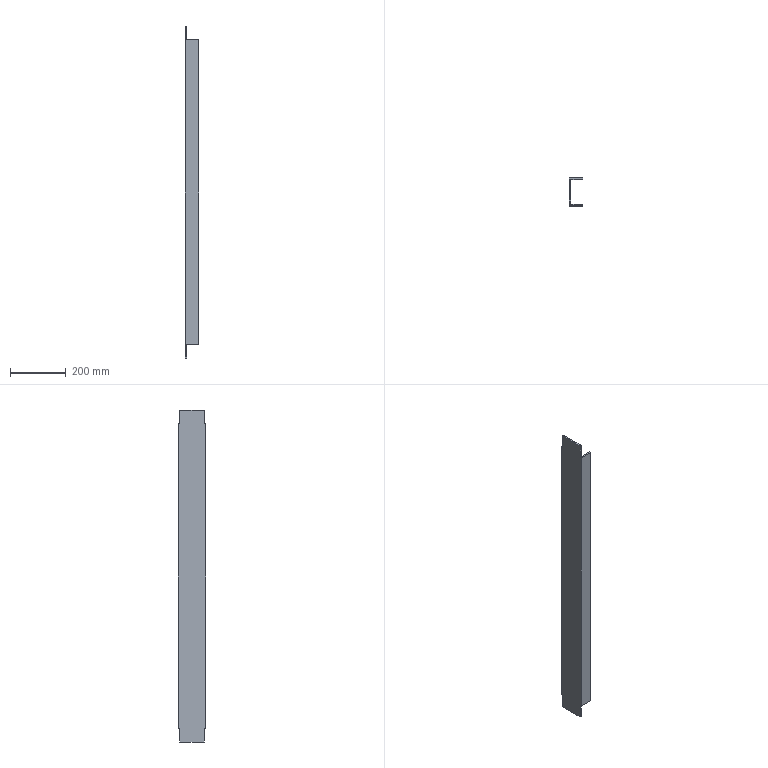Component | SolidWorks | 07ResistorBaseI-1 | 1 solid | 26 faces | box 48 x 100 x 1189 mm | volume 1154519 mm3 | plane 18 | cylinder 8 | commonest cylinder face diameters 12 x8
build123d program:
from build123d import *

# Parameters (mm, degrees)
EXTRUDE_THIN1_DEPTH            = 1189
SKETCH2_W                      = 48
SKETCH2_H                      = 50
CUT_EXTRUDE1_DEPTH             = 5.5
SKETCH3_W                      = 48
SKETCH3_H                      = 50
CUT_EXTRUDE2_DEPTH             = 5.5
F_12_0_12_DIAMETER_HOLE1_D     = 12
F_12_0_12_DIAMETER_HOLE1_DEPTH = 5.5


with BuildPart() as part:
    # Sketch1 → Extrude-Thin1 (new body)
    with BuildSketch(Plane.XY):
        Polygon((48, 0), (0, 0), (0, 100), (48, 100), (48, 94.5), (5.5, 94.5), (5.5, 5.5), (48, 5.5), align=None)
    extrude(amount=EXTRUDE_THIN1_DEPTH)

    # Sketch2 → Cut-Extrude1 (cut)
    with BuildSketch(Plane(origin=(0, 100, 0), x_dir=(1, 0, 0), z_dir=(0, 1, 0))):
        with Locations((24, -1164)):
            Rectangle(SKETCH2_W, SKETCH2_H)
        with Locations((24, -25)):
            Rectangle(SKETCH2_W, SKETCH2_H)
    extrude(amount=-CUT_EXTRUDE1_DEPTH, mode=Mode.SUBTRACT)

    # Sketch3 → Cut-Extrude2 (cut)
    with BuildSketch(Plane.XZ):
        with Locations((24, 25)):
            Rectangle(SKETCH3_W, SKETCH3_H)
        with Locations((24, 1164)):
            Rectangle(SKETCH3_W, SKETCH3_H)
    extrude(amount=-CUT_EXTRUDE2_DEPTH, mode=Mode.SUBTRACT)

    # 12.0 _12_ Diameter Hole1
    with Locations(Plane(origin=(0, 100, 0), x_dir=(-1, 0, 0), z_dir=(0, 1, 0))):
        with Locations((-25, 529.5), (-25, 659.5), (-25, 919.5), (-25, 269.5)):
            Hole(F_12_0_12_DIAMETER_HOLE1_D / 2, depth=F_12_0_12_DIAMETER_HOLE1_DEPTH)


solid = part.part

# Placed as in the assembly
solid = solid.moved(Location((2053.973, -139.54, 42.607), (0, 0, 0)))
STEP:
#1=CARTESIAN_POINT('',(81.849,-1.773,22.288));
#2=VERTEX_POINT('',#1);
#3=CARTESIAN_POINT('',(81.849,-1.773,22.76));
#4=VERTEX_POINT('',#3);
#5=CARTESIAN_POINT('',(81.849,-1.773,22.524));
#6=DIRECTION('',(0.,1.,0.));
#7=DIRECTION('',(0.,0.,1.));
#8=AXIS2_PLACEMENT_3D('',#5,#6,#7);
#9=CIRCLE('',#8,0.2362);
#10=EDGE_CURVE('',#2,#4,#9,.T.);
#11=ORIENTED_EDGE('',*,*,#10,.F.);
#12=CARTESIAN_POINT('',(81.849,-1.557,22.288));
#13=VERTEX_POINT('',#12);
#14=CARTESIAN_POINT('',(81.849,-1.557,22.288));
#15=DIRECTION('',(0.,1.,0.));
#16=VECTOR('',#15,39.37);
#17=LINE('',#14,#16);
#18=EDGE_CURVE('',#2,#13,#17,.T.);
#19=ORIENTED_EDGE('',*,*,#18,.T.);
#20=CARTESIAN_POINT('',(81.849,-1.557,22.76));
#21=VERTEX_POINT('',#20);
#22=CARTESIAN_POINT('',(81.849,-1.557,22.524));
#23=DIRECTION('',(0.,1.,0.));
#24=DIRECTION('',(0.,0.,1.));
#25=AXIS2_PLACEMENT_3D('',#22,#23,#24);
#26=CIRCLE('',#25,0.2362);
#27=EDGE_CURVE('',#13,#21,#26,.T.);
#28=ORIENTED_EDGE('',*,*,#27,.T.);
#29=CARTESIAN_POINT('',(81.849,-1.557,22.76));
#30=DIRECTION('',(0.,1.,0.));
#31=VECTOR('',#30,39.37);
#32=LINE('',#29,#31);
#33=EDGE_CURVE('',#4,#21,#32,.T.);
#34=ORIENTED_EDGE('',*,*,#33,.F.);
#35=EDGE_LOOP('',(#11,#19,#28,#34));
#36=FACE_OUTER_BOUND('',#35,.T.);
#37=CARTESIAN_POINT('',(81.849,-1.557,22.524));
#38=DIRECTION('',(0.,1.,0.));
#39=DIRECTION('',(0.,0.,1.));
#40=AXIS2_PLACEMENT_3D('',#37,#38,#39);
#41=CYLINDRICAL_SURFACE('',#40,0.2362);
#42=ADVANCED_FACE('',(#36),#41,.F.);
#43=CARTESIAN_POINT('',(81.849,-1.773,27.406));
#44=VERTEX_POINT('',#43);
#45=CARTESIAN_POINT('',(81.849,-1.773,27.878));
#46=VERTEX_POINT('',#45);
#47=CARTESIAN_POINT('',(81.849,-1.773,27.642));
#48=DIRECTION('',(0.,1.,0.));
#49=DIRECTION('',(0.,0.,1.));
#50=AXIS2_PLACEMENT_3D('',#47,#48,#49);
#51=CIRCLE('',#50,0.2362);
#52=EDGE_CURVE('',#44,#46,#51,.T.);
#53=ORIENTED_EDGE('',*,*,#52,.F.);
#54=CARTESIAN_POINT('',(81.849,-1.557,27.406));
#55=VERTEX_POINT('',#54);
#56=CARTESIAN_POINT('',(81.849,-1.557,27.406));
#57=DIRECTION('',(0.,1.,0.));
#58=VECTOR('',#57,39.37);
#59=LINE('',#56,#58);
#60=EDGE_CURVE('',#44,#55,#59,.T.);
#61=ORIENTED_EDGE('',*,*,#60,.T.);
#62=CARTESIAN_POINT('',(81.849,-1.557,27.878));
#63=VERTEX_POINT('',#62);
#64=CARTESIAN_POINT('',(81.849,-1.557,27.642));
#65=DIRECTION('',(0.,1.,0.));
#66=DIRECTION('',(0.,0.,1.));
#67=AXIS2_PLACEMENT_3D('',#64,#65,#66);
#68=CIRCLE('',#67,0.2362);
#69=EDGE_CURVE('',#55,#63,#68,.T.);
#70=ORIENTED_EDGE('',*,*,#69,.T.);
#71=CARTESIAN_POINT('',(81.849,-1.557,27.878));
#72=DIRECTION('',(0.,1.,0.));
#73=VECTOR('',#72,39.37);
#74=LINE('',#71,#73);
#75=EDGE_CURVE('',#46,#63,#74,.T.);
#76=ORIENTED_EDGE('',*,*,#75,.F.);
#77=EDGE_LOOP('',(#53,#61,#70,#76));
#78=FACE_OUTER_BOUND('',#77,.T.);
#79=CARTESIAN_POINT('',(81.849,-1.557,27.642));
#80=DIRECTION('',(0.,1.,0.));
#81=DIRECTION('',(0.,0.,1.));
#82=AXIS2_PLACEMENT_3D('',#79,#80,#81);
#83=CYLINDRICAL_SURFACE('',#82,0.2362);
#84=ADVANCED_FACE('',(#78),#83,.F.);
#85=CARTESIAN_POINT('',(81.849,-1.773,37.642));
#86=VERTEX_POINT('',#85);
#87=CARTESIAN_POINT('',(81.849,-1.773,38.114));
#88=VERTEX_POINT('',#87);
#89=CARTESIAN_POINT('',(81.849,-1.773,37.878));
#90=DIRECTION('',(0.,1.,0.));
#91=DIRECTION('',(0.,0.,1.));
#92=AXIS2_PLACEMENT_3D('',#89,#90,#91);
#93=CIRCLE('',#92,0.2362);
#94=EDGE_CURVE('',#86,#88,#93,.T.);
#95=ORIENTED_EDGE('',*,*,#94,.F.);
#96=CARTESIAN_POINT('',(81.849,-1.557,37.642));
#97=VERTEX_POINT('',#96);
#98=CARTESIAN_POINT('',(81.849,-1.557,37.642));
#99=DIRECTION('',(0.,1.,0.));
#100=VECTOR('',#99,39.37);
#101=LINE('',#98,#100);
#102=EDGE_CURVE('',#86,#97,#101,.T.);
#103=ORIENTED_EDGE('',*,*,#102,.T.);
#104=CARTESIAN_POINT('',(81.849,-1.557,38.114));
#105=VERTEX_POINT('',#104);
#106=CARTESIAN_POINT('',(81.849,-1.557,37.878));
#107=DIRECTION('',(0.,1.,0.));
#108=DIRECTION('',(0.,0.,1.));
#109=AXIS2_PLACEMENT_3D('',#106,#107,#108);
#110=CIRCLE('',#109,0.2362);
#111=EDGE_CURVE('',#97,#105,#110,.T.);
#112=ORIENTED_EDGE('',*,*,#111,.T.);
#113=CARTESIAN_POINT('',(81.849,-1.557,38.114));
#114=DIRECTION('',(0.,1.,0.));
#115=VECTOR('',#114,39.37);
#116=LINE('',#113,#115);
#117=EDGE_CURVE('',#88,#105,#116,.T.);
#118=ORIENTED_EDGE('',*,*,#117,.F.);
#119=EDGE_LOOP('',(#95,#103,#112,#118));
#120=FACE_OUTER_BOUND('',#119,.T.);
#121=CARTESIAN_POINT('',(81.849,-1.557,37.878));
#122=DIRECTION('',(0.,1.,0.));
#123=DIRECTION('',(0.,0.,1.));
#124=AXIS2_PLACEMENT_3D('',#121,#122,#123);
#125=CYLINDRICAL_SURFACE('',#124,0.2362);
#126=ADVANCED_FACE('',(#120),#125,.F.);
#127=CARTESIAN_POINT('',(81.849,-1.773,12.051));
#128=VERTEX_POINT('',#127);
#129=CARTESIAN_POINT('',(81.849,-1.773,12.524));
#130=VERTEX_POINT('',#129);
#131=CARTESIAN_POINT('',(81.849,-1.773,12.288));
#132=DIRECTION('',(0.,1.,0.));
#133=DIRECTION('',(0.,0.,1.));
#134=AXIS2_PLACEMENT_3D('',#131,#132,#133);
#135=CIRCLE('',#134,0.2362);
#136=EDGE_CURVE('',#128,#130,#135,.T.);
#137=ORIENTED_EDGE('',*,*,#136,.F.);
#138=CARTESIAN_POINT('',(81.849,-1.557,12.051));
#139=VERTEX_POINT('',#138);
#140=CARTESIAN_POINT('',(81.849,-1.557,12.051));
#141=DIRECTION('',(0.,1.,0.));
#142=VECTOR('',#141,39.37);
#143=LINE('',#140,#142);
#144=EDGE_CURVE('',#128,#139,#143,.T.);
#145=ORIENTED_EDGE('',*,*,#144,.T.);
#146=CARTESIAN_POINT('',(81.849,-1.557,12.524));
#147=VERTEX_POINT('',#146);
#148=CARTESIAN_POINT('',(81.849,-1.557,12.288));
#149=DIRECTION('',(0.,1.,0.));
#150=DIRECTION('',(0.,0.,1.));
#151=AXIS2_PLACEMENT_3D('',#148,#149,#150);
#152=CIRCLE('',#151,0.2362);
#153=EDGE_CURVE('',#139,#147,#152,.T.);
#154=ORIENTED_EDGE('',*,*,#153,.T.);
#155=CARTESIAN_POINT('',(81.849,-1.557,12.524));
#156=DIRECTION('',(0.,1.,0.));
#157=VECTOR('',#156,39.37);
#158=LINE('',#155,#157);
#159=EDGE_CURVE('',#130,#147,#158,.T.);
#160=ORIENTED_EDGE('',*,*,#159,.F.);
#161=EDGE_LOOP('',(#137,#145,#154,#160));
#162=FACE_OUTER_BOUND('',#161,.T.);
#163=CARTESIAN_POINT('',(81.849,-1.557,12.288));
#164=DIRECTION('',(0.,1.,0.));
#165=DIRECTION('',(0.,0.,1.));
#166=AXIS2_PLACEMENT_3D('',#163,#164,#165);
#167=CYLINDRICAL_SURFACE('',#166,0.2362);
#168=ADVANCED_FACE('',(#162),#167,.F.);
#169=CARTESIAN_POINT('',(80.865,-5.277,48.488));
#170=VERTEX_POINT('',#169);
#171=CARTESIAN_POINT('',(81.082,-5.277,48.488));
#172=VERTEX_POINT('',#171);
#173=CARTESIAN_POINT('',(82.755,-5.277,48.488));
#174=DIRECTION('',(1.,-0.,0.));
#175=VECTOR('',#174,39.37);
#176=LINE('',#173,#175);
#177=EDGE_CURVE('',#170,#172,#176,.T.);
#178=ORIENTED_EDGE('',*,*,#177,.T.);
#179=CARTESIAN_POINT('',(81.082,-1.773,48.488));
#180=VERTEX_POINT('',#179);
#181=CARTESIAN_POINT('',(81.082,-5.494,48.488));
#182=DIRECTION('',(0.,1.,0.));
#183=VECTOR('',#182,39.37);
#184=LINE('',#181,#183);
#185=EDGE_CURVE('',#172,#180,#184,.T.);
#186=ORIENTED_EDGE('',*,*,#185,.T.);
#187=CARTESIAN_POINT('',(80.865,-1.773,48.488));
#188=VERTEX_POINT('',#187);
#189=CARTESIAN_POINT('',(82.755,-1.773,48.488));
#190=DIRECTION('',(1.,0.,0.));
#191=VECTOR('',#190,39.37);
#192=LINE('',#189,#191);
#193=EDGE_CURVE('',#188,#180,#192,.T.);
#194=ORIENTED_EDGE('',*,*,#193,.F.);
#195=CARTESIAN_POINT('',(80.865,-5.494,48.488));
#196=DIRECTION('',(0.,1.,0.));
#197=VECTOR('',#196,39.37);
#198=LINE('',#195,#197);
#199=EDGE_CURVE('',#170,#188,#198,.T.);
#200=ORIENTED_EDGE('',*,*,#199,.F.);
#201=EDGE_LOOP('',(#178,#186,#194,#200));
#202=FACE_OUTER_BOUND('',#201,.T.);
#203=CARTESIAN_POINT('',(82.755,-1.773,48.488));
#204=DIRECTION('',(0.,0.,-1.));
#205=DIRECTION('',(-1.,0.,0.));
#206=AXIS2_PLACEMENT_3D('',#203,#204,#205);
#207=PLANE('',#206);
#208=ADVANCED_FACE('',(#202),#207,.F.);
#209=CARTESIAN_POINT('',(81.082,-5.277,1.677));
#210=VERTEX_POINT('',#209);
#211=CARTESIAN_POINT('',(81.082,-1.773,1.677));
#212=VERTEX_POINT('',#211);
#213=CARTESIAN_POINT('',(81.082,-5.494,1.677));
#214=DIRECTION('',(0.,1.,0.));
#215=VECTOR('',#214,39.37);
#216=LINE('',#213,#215);
#217=EDGE_CURVE('',#210,#212,#216,.T.);
#218=ORIENTED_EDGE('',*,*,#217,.F.);
#219=CARTESIAN_POINT('',(80.865,-5.277,1.677));
#220=VERTEX_POINT('',#219);
#221=CARTESIAN_POINT('',(82.755,-5.277,1.677));
#222=DIRECTION('',(-1.,0.,0.));
#223=VECTOR('',#222,39.37);
#224=LINE('',#221,#223);
#225=EDGE_CURVE('',#210,#220,#224,.T.);
#226=ORIENTED_EDGE('',*,*,#225,.T.);
#227=CARTESIAN_POINT('',(80.865,-1.773,1.677));
#228=VERTEX_POINT('',#227);
#229=CARTESIAN_POINT('',(80.865,-5.494,1.677));
#230=DIRECTION('',(0.,1.,0.));
#231=VECTOR('',#230,39.37);
#232=LINE('',#229,#231);
#233=EDGE_CURVE('',#220,#228,#232,.T.);
#234=ORIENTED_EDGE('',*,*,#233,.T.);
#235=CARTESIAN_POINT('',(82.755,-1.773,1.677));
#236=DIRECTION('',(1.,0.,0.));
#237=VECTOR('',#236,39.37);
#238=LINE('',#235,#237);
#239=EDGE_CURVE('',#228,#212,#238,.T.);
#240=ORIENTED_EDGE('',*,*,#239,.T.);
#241=EDGE_LOOP('',(#218,#226,#234,#240));
#242=FACE_OUTER_BOUND('',#241,.T.);
#243=CARTESIAN_POINT('',(82.755,-1.773,1.677));
#244=DIRECTION('',(0.,0.,-1.));
#245=DIRECTION('',(-1.,0.,0.));
#246=AXIS2_PLACEMENT_3D('',#243,#244,#245);
#247=PLANE('',#246);
#248=ADVANCED_FACE('',(#242),#247,.T.);
#249=CARTESIAN_POINT('',(81.849,-1.773,22.524));
#250=DIRECTION('',(0.,1.,0.));
#251=DIRECTION('',(0.,0.,1.));
#252=AXIS2_PLACEMENT_3D('',#249,#250,#251);
#253=CIRCLE('',#252,0.2362);
#254=EDGE_CURVE('',#4,#2,#253,.T.);
#255=ORIENTED_EDGE('',*,*,#254,.T.);
#256=ORIENTED_EDGE('',*,*,#10,.T.);
#257=EDGE_LOOP('',(#255,#256));
#258=FACE_BOUND('',#257,.T.);
#259=CARTESIAN_POINT('',(81.849,-1.773,27.642));
#260=DIRECTION('',(0.,1.,0.));
#261=DIRECTION('',(0.,0.,1.));
#262=AXIS2_PLACEMENT_3D('',#259,#260,#261);
#263=CIRCLE('',#262,0.2362);
#264=EDGE_CURVE('',#46,#44,#263,.T.);
#265=ORIENTED_EDGE('',*,*,#264,.T.);
#266=ORIENTED_EDGE('',*,*,#52,.T.);
#267=EDGE_LOOP('',(#265,#266));
#268=FACE_BOUND('',#267,.T.);
#269=CARTESIAN_POINT('',(81.849,-1.773,37.878));
#270=DIRECTION('',(0.,1.,0.));
#271=DIRECTION('',(0.,0.,1.));
#272=AXIS2_PLACEMENT_3D('',#269,#270,#271);
#273=CIRCLE('',#272,0.2362);
#274=EDGE_CURVE('',#88,#86,#273,.T.);
#275=ORIENTED_EDGE('',*,*,#274,.T.);
#276=ORIENTED_EDGE('',*,*,#94,.T.);
#277=EDGE_LOOP('',(#275,#276));
#278=FACE_BOUND('',#277,.T.);
#279=CARTESIAN_POINT('',(81.849,-1.773,12.288));
#280=DIRECTION('',(0.,1.,0.));
#281=DIRECTION('',(0.,0.,1.));
#282=AXIS2_PLACEMENT_3D('',#279,#280,#281);
#283=CIRCLE('',#282,0.2362);
#284=EDGE_CURVE('',#130,#128,#283,.T.);
#285=ORIENTED_EDGE('',*,*,#284,.T.);
#286=ORIENTED_EDGE('',*,*,#136,.T.);
#287=EDGE_LOOP('',(#285,#286));
#288=FACE_BOUND('',#287,.T.);
#289=CARTESIAN_POINT('',(81.082,-1.773,46.52));
#290=VERTEX_POINT('',#289);
#291=CARTESIAN_POINT('',(81.082,-1.773,3.646));
#292=VERTEX_POINT('',#291);
#293=CARTESIAN_POINT('',(81.082,-1.773,48.488));
#294=DIRECTION('',(0.,0.,-1.));
#295=VECTOR('',#294,39.37);
#296=LINE('',#293,#295);
#297=EDGE_CURVE('',#290,#292,#296,.T.);
#298=ORIENTED_EDGE('',*,*,#297,.T.);
#299=CARTESIAN_POINT('',(82.755,-1.773,3.646));
#300=VERTEX_POINT('',#299);
#301=CARTESIAN_POINT('',(82.755,-1.773,3.646));
#302=DIRECTION('',(-1.,0.,0.));
#303=VECTOR('',#302,39.37);
#304=LINE('',#301,#303);
#305=EDGE_CURVE('',#300,#292,#304,.T.);
#306=ORIENTED_EDGE('',*,*,#305,.F.);
#307=CARTESIAN_POINT('',(82.755,-1.773,46.52));
#308=VERTEX_POINT('',#307);
#309=CARTESIAN_POINT('',(82.755,-1.773,48.488));
#310=DIRECTION('',(0.,0.,-1.));
#311=VECTOR('',#310,39.37);
#312=LINE('',#309,#311);
#313=EDGE_CURVE('',#308,#300,#312,.T.);
#314=ORIENTED_EDGE('',*,*,#313,.F.);
#315=CARTESIAN_POINT('',(82.755,-1.773,46.52));
#316=DIRECTION('',(1.,0.,0.));
#317=VECTOR('',#316,39.37);
#318=LINE('',#315,#317);
#319=EDGE_CURVE('',#290,#308,#318,.T.);
#320=ORIENTED_EDGE('',*,*,#319,.F.);
#321=EDGE_LOOP('',(#298,#306,#314,#320));
#322=FACE_OUTER_BOUND('',#321,.T.);
#323=CARTESIAN_POINT('',(80.865,-1.773,48.488));
#324=DIRECTION('',(0.,1.,0.));
#325=DIRECTION('',(0.,0.,1.));
#326=AXIS2_PLACEMENT_3D('',#323,#324,#325);
#327=PLANE('',#326);
#328=ADVANCED_FACE('',(#258,#268,#278,#288,#322),#327,.F.);
#329=CARTESIAN_POINT('',(82.755,-1.557,3.646));
#330=VERTEX_POINT('',#329);
#331=CARTESIAN_POINT('',(82.755,-4.502,3.646));
#332=DIRECTION('',(0.,1.,0.));
#333=VECTOR('',#332,39.37);
#334=LINE('',#331,#333);
#335=EDGE_CURVE('',#300,#330,#334,.T.);
#336=ORIENTED_EDGE('',*,*,#335,.T.);
#337=CARTESIAN_POINT('',(82.755,-1.557,46.52));
#338=VERTEX_POINT('',#337);
#339=CARTESIAN_POINT('',(82.755,-1.557,48.488));
#340=DIRECTION('',(0.,0.,-1.));
#341=VECTOR('',#340,39.37);
#342=LINE('',#339,#341);
#343=EDGE_CURVE('',#338,#330,#342,.T.);
#344=ORIENTED_EDGE('',*,*,#343,.F.);
#345=CARTESIAN_POINT('',(82.755,-4.502,46.52));
#346=DIRECTION('',(0.,1.,0.));
#347=VECTOR('',#346,39.37);
#348=LINE('',#345,#347);
#349=EDGE_CURVE('',#308,#338,#348,.T.);
#350=ORIENTED_EDGE('',*,*,#349,.F.);
#351=ORIENTED_EDGE('',*,*,#313,.T.);
#352=EDGE_LOOP('',(#336,#344,#350,#351));
#353=FACE_OUTER_BOUND('',#352,.T.);
#354=CARTESIAN_POINT('',(82.755,-1.557,48.488));
#355=DIRECTION('',(1.,0.,0.));
#356=DIRECTION('',(0.,0.,-1.));
#357=AXIS2_PLACEMENT_3D('',#354,#355,#356);
#358=PLANE('',#357);
#359=ADVANCED_FACE('',(#353),#358,.T.);
#360=CARTESIAN_POINT('',(81.849,-1.557,22.524));
#361=DIRECTION('',(0.,1.,0.));
#362=DIRECTION('',(0.,0.,1.));
#363=AXIS2_PLACEMENT_3D('',#360,#361,#362);
#364=CIRCLE('',#363,0.2362);
#365=EDGE_CURVE('',#21,#13,#364,.T.);
#366=ORIENTED_EDGE('',*,*,#365,.F.);
#367=ORIENTED_EDGE('',*,*,#27,.F.);
#368=EDGE_LOOP('',(#366,#367));
#369=FACE_BOUND('',#368,.T.);
#370=CARTESIAN_POINT('',(81.849,-1.557,27.642));
#371=DIRECTION('',(0.,1.,0.));
#372=DIRECTION('',(0.,0.,1.));
#373=AXIS2_PLACEMENT_3D('',#370,#371,#372);
#374=CIRCLE('',#373,0.2362);
#375=EDGE_CURVE('',#63,#55,#374,.T.);
#376=ORIENTED_EDGE('',*,*,#375,.F.);
#377=ORIENTED_EDGE('',*,*,#69,.F.);
#378=EDGE_LOOP('',(#376,#377));
#379=FACE_BOUND('',#378,.T.);
#380=CARTESIAN_POINT('',(81.849,-1.557,37.878));
#381=DIRECTION('',(0.,1.,0.));
#382=DIRECTION('',(0.,0.,1.));
#383=AXIS2_PLACEMENT_3D('',#380,#381,#382);
#384=CIRCLE('',#383,0.2362);
#385=EDGE_CURVE('',#105,#97,#384,.T.);
#386=ORIENTED_EDGE('',*,*,#385,.F.);
#387=ORIENTED_EDGE('',*,*,#111,.F.);
#388=EDGE_LOOP('',(#386,#387));
#389=FACE_BOUND('',#388,.T.);
#390=CARTESIAN_POINT('',(81.849,-1.557,12.288));
#391=DIRECTION('',(0.,1.,0.));
#392=DIRECTION('',(0.,0.,1.));
#393=AXIS2_PLACEMENT_3D('',#390,#391,#392);
#394=CIRCLE('',#393,0.2362);
#395=EDGE_CURVE('',#147,#139,#394,.T.);
#396=ORIENTED_EDGE('',*,*,#395,.F.);
#397=ORIENTED_EDGE('',*,*,#153,.F.);
#398=EDGE_LOOP('',(#396,#397));
#399=FACE_BOUND('',#398,.T.);
#400=CARTESIAN_POINT('',(80.865,-1.557,3.646));
#401=VERTEX_POINT('',#400);
#402=CARTESIAN_POINT('',(82.755,-1.557,3.646));
#403=DIRECTION('',(1.,0.,0.));
#404=VECTOR('',#403,39.37);
#405=LINE('',#402,#404);
#406=EDGE_CURVE('',#401,#330,#405,.T.);
#407=ORIENTED_EDGE('',*,*,#406,.F.);
#408=CARTESIAN_POINT('',(80.865,-1.557,46.52));
#409=VERTEX_POINT('',#408);
#410=CARTESIAN_POINT('',(80.865,-1.557,48.488));
#411=DIRECTION('',(0.,0.,-1.));
#412=VECTOR('',#411,39.37);
#413=LINE('',#410,#412);
#414=EDGE_CURVE('',#409,#401,#413,.T.);
#415=ORIENTED_EDGE('',*,*,#414,.F.);
#416=CARTESIAN_POINT('',(82.755,-1.557,46.52));
#417=DIRECTION('',(-1.,0.,0.));
#418=VECTOR('',#417,39.37);
#419=LINE('',#416,#418);
#420=EDGE_CURVE('',#338,#409,#419,.T.);
#421=ORIENTED_EDGE('',*,*,#420,.F.);
#422=ORIENTED_EDGE('',*,*,#343,.T.);
#423=EDGE_LOOP('',(#407,#415,#421,#422));
#424=FACE_OUTER_BOUND('',#423,.T.);
#425=CARTESIAN_POINT('',(80.865,-1.557,48.488));
#426=DIRECTION('',(0.,1.,0.));
#427=DIRECTION('',(0.,0.,1.));
#428=AXIS2_PLACEMENT_3D('',#425,#426,#427);
#429=PLANE('',#428);
#430=ADVANCED_FACE('',(#369,#379,#389,#399,#424),#429,.T.);
#431=CARTESIAN_POINT('',(80.865,-5.277,46.52));
#432=VERTEX_POINT('',#431);
#433=CARTESIAN_POINT('',(80.865,-5.494,46.52));
#434=VERTEX_POINT('',#433);
#435=CARTESIAN_POINT('',(80.865,-2.548,46.52));
#436=DIRECTION('',(-0.,-1.,0.));
#437=VECTOR('',#436,39.37);
#438=LINE('',#435,#437);
#439=EDGE_CURVE('',#432,#434,#438,.T.);
#440=ORIENTED_EDGE('',*,*,#439,.F.);
#441=CARTESIAN_POINT('',(80.865,-5.277,48.488));
#442=DIRECTION('',(0.,0.,1.));
#443=VECTOR('',#442,39.37);
#444=LINE('',#441,#443);
#445=EDGE_CURVE('',#432,#170,#444,.T.);
#446=ORIENTED_EDGE('',*,*,#445,.T.);
#447=ORIENTED_EDGE('',*,*,#199,.T.);
#448=CARTESIAN_POINT('',(80.865,-1.773,46.52));
#449=VERTEX_POINT('',#448);
#450=CARTESIAN_POINT('',(80.865,-1.773,48.488));
#451=DIRECTION('',(0.,0.,-1.));
#452=VECTOR('',#451,39.37);
#453=LINE('',#450,#452);
#454=EDGE_CURVE('',#188,#449,#453,.T.);
#455=ORIENTED_EDGE('',*,*,#454,.T.);
#456=CARTESIAN_POINT('',(80.865,-4.502,46.52));
#457=DIRECTION('',(0.,1.,0.));
#458=VECTOR('',#457,39.37);
#459=LINE('',#456,#458);
#460=EDGE_CURVE('',#449,#409,#459,.T.);
#461=ORIENTED_EDGE('',*,*,#460,.T.);
#462=ORIENTED_EDGE('',*,*,#414,.T.);
#463=CARTESIAN_POINT('',(80.865,-1.773,3.646));
#464=VERTEX_POINT('',#463);
#465=CARTESIAN_POINT('',(80.865,-4.502,3.646));
#466=DIRECTION('',(0.,1.,0.));
#467=VECTOR('',#466,39.37);
#468=LINE('',#465,#467);
#469=EDGE_CURVE('',#464,#401,#468,.T.);
#470=ORIENTED_EDGE('',*,*,#469,.F.);
#471=CARTESIAN_POINT('',(80.865,-1.773,1.677));
#472=DIRECTION('',(0.,0.,-1.));
#473=VECTOR('',#472,39.37);
#474=LINE('',#471,#473);
#475=EDGE_CURVE('',#464,#228,#474,.T.);
#476=ORIENTED_EDGE('',*,*,#475,.T.);
#477=ORIENTED_EDGE('',*,*,#233,.F.);
#478=CARTESIAN_POINT('',(80.865,-5.277,3.646));
#479=VERTEX_POINT('',#478);
#480=CARTESIAN_POINT('',(80.865,-5.277,1.677));
#481=DIRECTION('',(0.,0.,1.));
#482=VECTOR('',#481,39.37);
#483=LINE('',#480,#482);
#484=EDGE_CURVE('',#220,#479,#483,.T.);
#485=ORIENTED_EDGE('',*,*,#484,.T.);
#486=CARTESIAN_POINT('',(80.865,-5.494,3.646));
#487=VERTEX_POINT('',#486);
#488=CARTESIAN_POINT('',(80.865,-2.548,3.646));
#489=DIRECTION('',(-0.,-1.,0.));
#490=VECTOR('',#489,39.37);
#491=LINE('',#488,#490);
#492=EDGE_CURVE('',#479,#487,#491,.T.);
#493=ORIENTED_EDGE('',*,*,#492,.T.);
#494=CARTESIAN_POINT('',(80.865,-5.494,48.488));
#495=DIRECTION('',(0.,0.,-1.));
#496=VECTOR('',#495,39.37);
#497=LINE('',#494,#496);
#498=EDGE_CURVE('',#434,#487,#497,.T.);
#499=ORIENTED_EDGE('',*,*,#498,.F.);
#500=EDGE_LOOP('',(#440,#446,#447,#455,#461,#462,#470,#476,#477,#485,#493,#499));
#501=FACE_OUTER_BOUND('',#500,.T.);
#502=CARTESIAN_POINT('',(80.865,-5.494,48.488));
#503=DIRECTION('',(-1.,0.,0.));
#504=DIRECTION('',(0.,0.,1.));
#505=AXIS2_PLACEMENT_3D('',#502,#503,#504);
#506=PLANE('',#505);
#507=ADVANCED_FACE('',(#501),#506,.T.);
#508=CARTESIAN_POINT('',(82.755,-5.494,46.52));
#509=VERTEX_POINT('',#508);
#510=CARTESIAN_POINT('',(82.755,-5.494,46.52));
#511=DIRECTION('',(1.,-0.,0.));
#512=VECTOR('',#511,39.37);
#513=LINE('',#510,#512);
#514=EDGE_CURVE('',#434,#509,#513,.T.);
#515=ORIENTED_EDGE('',*,*,#514,.F.);
#516=ORIENTED_EDGE('',*,*,#498,.T.);
#517=CARTESIAN_POINT('',(82.755,-5.494,3.646));
#518=VERTEX_POINT('',#517);
#519=CARTESIAN_POINT('',(82.755,-5.494,3.646));
#520=DIRECTION('',(-1.,0.,0.));
#521=VECTOR('',#520,39.37);
#522=LINE('',#519,#521);
#523=EDGE_CURVE('',#518,#487,#522,.T.);
#524=ORIENTED_EDGE('',*,*,#523,.F.);
#525=CARTESIAN_POINT('',(82.755,-5.494,48.488));
#526=DIRECTION('',(0.,0.,-1.));
#527=VECTOR('',#526,39.37);
#528=LINE('',#525,#527);
#529=EDGE_CURVE('',#509,#518,#528,.T.);
#530=ORIENTED_EDGE('',*,*,#529,.F.);
#531=EDGE_LOOP('',(#515,#516,#524,#530));
#532=FACE_OUTER_BOUND('',#531,.T.);
#533=CARTESIAN_POINT('',(82.755,-5.494,48.488));
#534=DIRECTION('',(-0.,-1.,0.));
#535=DIRECTION('',(1.,-0.,0.));
#536=AXIS2_PLACEMENT_3D('',#533,#534,#535);
#537=PLANE('',#536);
#538=ADVANCED_FACE('',(#532),#537,.T.);
#539=CARTESIAN_POINT('',(82.755,-5.277,46.52));
#540=VERTEX_POINT('',#539);
#541=CARTESIAN_POINT('',(82.755,-2.548,46.52));
#542=DIRECTION('',(-0.,-1.,0.));
#543=VECTOR('',#542,39.37);
#544=LINE('',#541,#543);
#545=EDGE_CURVE('',#540,#509,#544,.T.);
#546=ORIENTED_EDGE('',*,*,#545,.T.);
#547=ORIENTED_EDGE('',*,*,#529,.T.);
#548=CARTESIAN_POINT('',(82.755,-5.277,3.646));
#549=VERTEX_POINT('',#548);
#550=CARTESIAN_POINT('',(82.755,-2.548,3.646));
#551=DIRECTION('',(-0.,-1.,0.));
#552=VECTOR('',#551,39.37);
#553=LINE('',#550,#552);
#554=EDGE_CURVE('',#549,#518,#553,.T.);
#555=ORIENTED_EDGE('',*,*,#554,.F.);
#556=CARTESIAN_POINT('',(82.755,-5.277,48.488));
#557=DIRECTION('',(0.,0.,-1.));
#558=VECTOR('',#557,39.37);
#559=LINE('',#556,#558);
#560=EDGE_CURVE('',#540,#549,#559,.T.);
#561=ORIENTED_EDGE('',*,*,#560,.F.);
#562=EDGE_LOOP('',(#546,#547,#555,#561));
#563=FACE_OUTER_BOUND('',#562,.T.);
#564=CARTESIAN_POINT('',(82.755,-5.277,48.488));
#565=DIRECTION('',(1.,0.,0.));
#566=DIRECTION('',(0.,0.,-1.));
#567=AXIS2_PLACEMENT_3D('',#564,#565,#566);
#568=PLANE('',#567);
#569=ADVANCED_FACE('',(#563),#568,.T.);
#570=CARTESIAN_POINT('',(81.082,-5.277,46.52));
#571=VERTEX_POINT('',#570);
#572=CARTESIAN_POINT('',(81.082,-5.277,3.646));
#573=VERTEX_POINT('',#572);
#574=CARTESIAN_POINT('',(81.082,-5.277,48.488));
#575=DIRECTION('',(0.,0.,-1.));
#576=VECTOR('',#575,39.37);
#577=LINE('',#574,#576);
#578=EDGE_CURVE('',#571,#573,#577,.T.);
#579=ORIENTED_EDGE('',*,*,#578,.F.);
#580=CARTESIAN_POINT('',(82.755,-5.277,46.52));
#581=DIRECTION('',(-1.,0.,0.));
#582=VECTOR('',#581,39.37);
#583=LINE('',#580,#582);
#584=EDGE_CURVE('',#540,#571,#583,.T.);
#585=ORIENTED_EDGE('',*,*,#584,.F.);
#586=ORIENTED_EDGE('',*,*,#560,.T.);
#587=CARTESIAN_POINT('',(82.755,-5.277,3.646));
#588=DIRECTION('',(1.,-0.,0.));
#589=VECTOR('',#588,39.37);
#590=LINE('',#587,#589);
#591=EDGE_CURVE('',#573,#549,#590,.T.);
#592=ORIENTED_EDGE('',*,*,#591,.F.);
#593=EDGE_LOOP('',(#579,#585,#586,#592));
#594=FACE_OUTER_BOUND('',#593,.T.);
#595=CARTESIAN_POINT('',(82.755,-5.277,48.488));
#596=DIRECTION('',(-0.,-1.,0.));
#597=DIRECTION('',(1.,-0.,0.));
#598=AXIS2_PLACEMENT_3D('',#595,#596,#597);
#599=PLANE('',#598);
#600=ADVANCED_FACE('',(#594),#599,.F.);
#601=ORIENTED_EDGE('',*,*,#217,.T.);
#602=CARTESIAN_POINT('',(81.082,-1.773,48.488));
#603=DIRECTION('',(0.,0.,-1.));
#604=VECTOR('',#603,39.37);
#605=LINE('',#602,#604);
#606=EDGE_CURVE('',#292,#212,#605,.T.);
#607=ORIENTED_EDGE('',*,*,#606,.F.);
#608=ORIENTED_EDGE('',*,*,#297,.F.);
#609=CARTESIAN_POINT('',(81.082,-1.773,48.488));
#610=DIRECTION('',(0.,0.,-1.));
#611=VECTOR('',#610,39.37);
#612=LINE('',#609,#611);
#613=EDGE_CURVE('',#180,#290,#612,.T.);
#614=ORIENTED_EDGE('',*,*,#613,.F.);
#615=ORIENTED_EDGE('',*,*,#185,.F.);
#616=CARTESIAN_POINT('',(81.082,-5.277,48.488));
#617=DIRECTION('',(0.,0.,-1.));
#618=VECTOR('',#617,39.37);
#619=LINE('',#616,#618);
#620=EDGE_CURVE('',#172,#571,#619,.T.);
#621=ORIENTED_EDGE('',*,*,#620,.T.);
#622=ORIENTED_EDGE('',*,*,#578,.T.);
#623=CARTESIAN_POINT('',(81.082,-5.277,48.488));
#624=DIRECTION('',(0.,0.,-1.));
#625=VECTOR('',#624,39.37);
#626=LINE('',#623,#625);
#627=EDGE_CURVE('',#573,#210,#626,.T.);
#628=ORIENTED_EDGE('',*,*,#627,.T.);
#629=EDGE_LOOP('',(#601,#607,#608,#614,#615,#621,#622,#628));
#630=FACE_OUTER_BOUND('',#629,.T.);
#631=CARTESIAN_POINT('',(81.082,-5.494,48.488));
#632=DIRECTION('',(-1.,0.,0.));
#633=DIRECTION('',(0.,0.,1.));
#634=AXIS2_PLACEMENT_3D('',#631,#632,#633);
#635=PLANE('',#634);
#636=ADVANCED_FACE('',(#630),#635,.F.);
#637=ORIENTED_EDGE('',*,*,#613,.T.);
#638=CARTESIAN_POINT('',(82.755,-1.773,46.52));
#639=DIRECTION('',(1.,0.,0.));
#640=VECTOR('',#639,39.37);
#641=LINE('',#638,#640);
#642=EDGE_CURVE('',#449,#290,#641,.T.);
#643=ORIENTED_EDGE('',*,*,#642,.F.);
#644=ORIENTED_EDGE('',*,*,#454,.F.);
#645=ORIENTED_EDGE('',*,*,#193,.T.);
#646=EDGE_LOOP('',(#637,#643,#644,#645));
#647=FACE_OUTER_BOUND('',#646,.T.);
#648=CARTESIAN_POINT('',(80.865,-1.773,48.488));
#649=DIRECTION('',(0.,1.,0.));
#650=DIRECTION('',(0.,0.,1.));
#651=AXIS2_PLACEMENT_3D('',#648,#649,#650);
#652=PLANE('',#651);
#653=ADVANCED_FACE('',(#647),#652,.T.);
#654=ORIENTED_EDGE('',*,*,#642,.T.);
#655=ORIENTED_EDGE('',*,*,#319,.T.);
#656=ORIENTED_EDGE('',*,*,#349,.T.);
#657=ORIENTED_EDGE('',*,*,#420,.T.);
#658=ORIENTED_EDGE('',*,*,#460,.F.);
#659=EDGE_LOOP('',(#654,#655,#656,#657,#658));
#660=FACE_OUTER_BOUND('',#659,.T.);
#661=CARTESIAN_POINT('',(82.755,-4.502,46.52));
#662=DIRECTION('',(0.,0.,-1.));
#663=DIRECTION('',(-1.,0.,0.));
#664=AXIS2_PLACEMENT_3D('',#661,#662,#663);
#665=PLANE('',#664);
#666=ADVANCED_FACE('',(#660),#665,.F.);
#667=ORIENTED_EDGE('',*,*,#606,.T.);
#668=ORIENTED_EDGE('',*,*,#239,.F.);
#669=ORIENTED_EDGE('',*,*,#475,.F.);
#670=CARTESIAN_POINT('',(82.755,-1.773,3.646));
#671=DIRECTION('',(-1.,0.,0.));
#672=VECTOR('',#671,39.37);
#673=LINE('',#670,#672);
#674=EDGE_CURVE('',#292,#464,#673,.T.);
#675=ORIENTED_EDGE('',*,*,#674,.F.);
#676=EDGE_LOOP('',(#667,#668,#669,#675));
#677=FACE_OUTER_BOUND('',#676,.T.);
#678=CARTESIAN_POINT('',(80.865,-1.773,48.488));
#679=DIRECTION('',(0.,1.,0.));
#680=DIRECTION('',(0.,0.,1.));
#681=AXIS2_PLACEMENT_3D('',#678,#679,#680);
#682=PLANE('',#681);
#683=ADVANCED_FACE('',(#677),#682,.T.);
#684=ORIENTED_EDGE('',*,*,#305,.T.);
#685=ORIENTED_EDGE('',*,*,#674,.T.);
#686=ORIENTED_EDGE('',*,*,#469,.T.);
#687=ORIENTED_EDGE('',*,*,#406,.T.);
#688=ORIENTED_EDGE('',*,*,#335,.F.);
#689=EDGE_LOOP('',(#684,#685,#686,#687,#688));
#690=FACE_OUTER_BOUND('',#689,.T.);
#691=CARTESIAN_POINT('',(82.755,-4.502,3.646));
#692=DIRECTION('',(0.,0.,1.));
#693=DIRECTION('',(1.,0.,0.));
#694=AXIS2_PLACEMENT_3D('',#691,#692,#693);
#695=PLANE('',#694);
#696=ADVANCED_FACE('',(#690),#695,.F.);
#697=ORIENTED_EDGE('',*,*,#627,.F.);
#698=CARTESIAN_POINT('',(82.755,-5.277,3.646));
#699=DIRECTION('',(1.,-0.,0.));
#700=VECTOR('',#699,39.37);
#701=LINE('',#698,#700);
#702=EDGE_CURVE('',#479,#573,#701,.T.);
#703=ORIENTED_EDGE('',*,*,#702,.F.);
#704=ORIENTED_EDGE('',*,*,#484,.F.);
#705=ORIENTED_EDGE('',*,*,#225,.F.);
#706=EDGE_LOOP('',(#697,#703,#704,#705));
#707=FACE_OUTER_BOUND('',#706,.T.);
#708=CARTESIAN_POINT('',(82.755,-5.277,48.488));
#709=DIRECTION('',(-0.,-1.,0.));
#710=DIRECTION('',(1.,-0.,0.));
#711=AXIS2_PLACEMENT_3D('',#708,#709,#710);
#712=PLANE('',#711);
#713=ADVANCED_FACE('',(#707),#712,.T.);
#714=ORIENTED_EDGE('',*,*,#702,.T.);
#715=ORIENTED_EDGE('',*,*,#591,.T.);
#716=ORIENTED_EDGE('',*,*,#554,.T.);
#717=ORIENTED_EDGE('',*,*,#523,.T.);
#718=ORIENTED_EDGE('',*,*,#492,.F.);
#719=EDGE_LOOP('',(#714,#715,#716,#717,#718));
#720=FACE_OUTER_BOUND('',#719,.T.);
#721=CARTESIAN_POINT('',(82.755,-2.548,3.646));
#722=DIRECTION('',(0.,0.,1.));
#723=DIRECTION('',(1.,0.,0.));
#724=AXIS2_PLACEMENT_3D('',#721,#722,#723);
#725=PLANE('',#724);
#726=ADVANCED_FACE('',(#720),#725,.F.);
#727=ORIENTED_EDGE('',*,*,#620,.F.);
#728=ORIENTED_EDGE('',*,*,#177,.F.);
#729=ORIENTED_EDGE('',*,*,#445,.F.);
#730=CARTESIAN_POINT('',(82.755,-5.277,46.52));
#731=DIRECTION('',(-1.,0.,0.));
#732=VECTOR('',#731,39.37);
#733=LINE('',#730,#732);
#734=EDGE_CURVE('',#571,#432,#733,.T.);
#735=ORIENTED_EDGE('',*,*,#734,.F.);
#736=EDGE_LOOP('',(#727,#728,#729,#735));
#737=FACE_OUTER_BOUND('',#736,.T.);
#738=CARTESIAN_POINT('',(82.755,-5.277,48.488));
#739=DIRECTION('',(-0.,-1.,0.));
#740=DIRECTION('',(1.,-0.,0.));
#741=AXIS2_PLACEMENT_3D('',#738,#739,#740);
#742=PLANE('',#741);
#743=ADVANCED_FACE('',(#737),#742,.T.);
#744=ORIENTED_EDGE('',*,*,#584,.T.);
#745=ORIENTED_EDGE('',*,*,#734,.T.);
#746=ORIENTED_EDGE('',*,*,#439,.T.);
#747=ORIENTED_EDGE('',*,*,#514,.T.);
#748=ORIENTED_EDGE('',*,*,#545,.F.);
#749=EDGE_LOOP('',(#744,#745,#746,#747,#748));
#750=FACE_OUTER_BOUND('',#749,.T.);
#751=CARTESIAN_POINT('',(82.755,-2.548,46.52));
#752=DIRECTION('',(0.,0.,-1.));
#753=DIRECTION('',(-1.,0.,0.));
#754=AXIS2_PLACEMENT_3D('',#751,#752,#753);
#755=PLANE('',#754);
#756=ADVANCED_FACE('',(#750),#755,.F.);
#757=ORIENTED_EDGE('',*,*,#144,.F.);
#758=ORIENTED_EDGE('',*,*,#284,.F.);
#759=ORIENTED_EDGE('',*,*,#159,.T.);
#760=ORIENTED_EDGE('',*,*,#395,.T.);
#761=EDGE_LOOP('',(#757,#758,#759,#760));
#762=FACE_OUTER_BOUND('',#761,.T.);
#763=CARTESIAN_POINT('',(81.849,-1.557,12.288));
#764=DIRECTION('',(0.,1.,0.));
#765=DIRECTION('',(0.,0.,1.));
#766=AXIS2_PLACEMENT_3D('',#763,#764,#765);
#767=CYLINDRICAL_SURFACE('',#766,0.2362);
#768=ADVANCED_FACE('',(#762),#767,.F.);
#769=ORIENTED_EDGE('',*,*,#102,.F.);
#770=ORIENTED_EDGE('',*,*,#274,.F.);
#771=ORIENTED_EDGE('',*,*,#117,.T.);
#772=ORIENTED_EDGE('',*,*,#385,.T.);
#773=EDGE_LOOP('',(#769,#770,#771,#772));
#774=FACE_OUTER_BOUND('',#773,.T.);
#775=CARTESIAN_POINT('',(81.849,-1.557,37.878));
#776=DIRECTION('',(0.,1.,0.));
#777=DIRECTION('',(0.,0.,1.));
#778=AXIS2_PLACEMENT_3D('',#775,#776,#777);
#779=CYLINDRICAL_SURFACE('',#778,0.2362);
#780=ADVANCED_FACE('',(#774),#779,.F.);
#781=ORIENTED_EDGE('',*,*,#60,.F.);
#782=ORIENTED_EDGE('',*,*,#264,.F.);
#783=ORIENTED_EDGE('',*,*,#75,.T.);
#784=ORIENTED_EDGE('',*,*,#375,.T.);
#785=EDGE_LOOP('',(#781,#782,#783,#784));
#786=FACE_OUTER_BOUND('',#785,.T.);
#787=CARTESIAN_POINT('',(81.849,-1.557,27.642));
#788=DIRECTION('',(0.,1.,0.));
#789=DIRECTION('',(0.,0.,1.));
#790=AXIS2_PLACEMENT_3D('',#787,#788,#789);
#791=CYLINDRICAL_SURFACE('',#790,0.2362);
#792=ADVANCED_FACE('',(#786),#791,.F.);
#793=ORIENTED_EDGE('',*,*,#18,.F.);
#794=ORIENTED_EDGE('',*,*,#254,.F.);
#795=ORIENTED_EDGE('',*,*,#33,.T.);
#796=ORIENTED_EDGE('',*,*,#365,.T.);
#797=EDGE_LOOP('',(#793,#794,#795,#796));
#798=FACE_OUTER_BOUND('',#797,.T.);
#799=CARTESIAN_POINT('',(81.849,-1.557,22.524));
#800=DIRECTION('',(0.,1.,0.));
#801=DIRECTION('',(0.,0.,1.));
#802=AXIS2_PLACEMENT_3D('',#799,#800,#801);
#803=CYLINDRICAL_SURFACE('',#802,0.2362);
#804=ADVANCED_FACE('',(#798),#803,.F.);
#805=CLOSED_SHELL('',(#42,#84,#126,#168,#208,#248,#328,#359,#430,#507,#538,#569,#600,#636,#653,#666,#683,#696,#713,#726,#743,#756,#768,#780,#792,#804));
#806=MANIFOLD_SOLID_BREP('',#805);
#807=CARTESIAN_POINT('',(0.,0.,0.));
#808=DIRECTION('',(0.,0.,1.));
#809=DIRECTION('',(1.,0.,0.));
#810=AXIS2_PLACEMENT_3D('',#807,#808,#809);
#811=(LENGTH_UNIT()NAMED_UNIT(*)SI_UNIT($,.METRE.));
#812=LENGTH_MEASURE_WITH_UNIT(LENGTH_MEASURE(0.0254),#811);
#813=DIMENSIONAL_EXPONENTS(1.,0.,0.,0.,0.,0.,0.);
#814=(CONVERSION_BASED_UNIT('',#812)LENGTH_UNIT()NAMED_UNIT(#813));
#815=UNCERTAINTY_MEASURE_WITH_UNIT(LENGTH_MEASURE(0.00001),#814,'','');
#816=(NAMED_UNIT(*)PLANE_ANGLE_UNIT()SI_UNIT($,.RADIAN.));
#817=(NAMED_UNIT(*)SI_UNIT($,.STERADIAN.)SOLID_ANGLE_UNIT());
#818=(GEOMETRIC_REPRESENTATION_CONTEXT(3)GLOBAL_UNCERTAINTY_ASSIGNED_CONTEXT((#815))GLOBAL_UNIT_ASSIGNED_CONTEXT((#814,#816,#817))REPRESENTATION_CONTEXT('',''));
#819=ADVANCED_BREP_SHAPE_REPRESENTATION('',(#806,#810),#818);
#820=COLOUR_RGB('',0.7922,0.8196,0.9333);
#821=FILL_AREA_STYLE_COLOUR('',#820);
#822=FILL_AREA_STYLE('',(#821));
#823=SURFACE_STYLE_FILL_AREA(#822);
#824=SURFACE_SIDE_STYLE('',(#823));
#825=SURFACE_STYLE_USAGE(.BOTH.,#824);
#826=PRESENTATION_STYLE_ASSIGNMENT((#825));
#827=STYLED_ITEM('',(#826),#806);
#828=(LENGTH_UNIT()NAMED_UNIT(*)SI_UNIT($,.METRE.));
#829=LENGTH_MEASURE_WITH_UNIT(LENGTH_MEASURE(0.0254),#828);
#830=DIMENSIONAL_EXPONENTS(1.,0.,0.,0.,0.,0.,0.);
#831=(CONVERSION_BASED_UNIT('',#829)LENGTH_UNIT()NAMED_UNIT(#830));
#832=UNCERTAINTY_MEASURE_WITH_UNIT(LENGTH_MEASURE(0.00001),#831,'','');
#833=(NAMED_UNIT(*)PLANE_ANGLE_UNIT()SI_UNIT($,.RADIAN.));
#834=(NAMED_UNIT(*)SI_UNIT($,.STERADIAN.)SOLID_ANGLE_UNIT());
#835=(GEOMETRIC_REPRESENTATION_CONTEXT(3)GLOBAL_UNCERTAINTY_ASSIGNED_CONTEXT((#832))GLOBAL_UNIT_ASSIGNED_CONTEXT((#831,#833,#834))REPRESENTATION_CONTEXT('',''));
#836=MECHANICAL_DESIGN_GEOMETRIC_PRESENTATION_REPRESENTATION('',(#827),#835);
#837=PRESENTATION_LAYER_ASSIGNMENT('','',(#827));